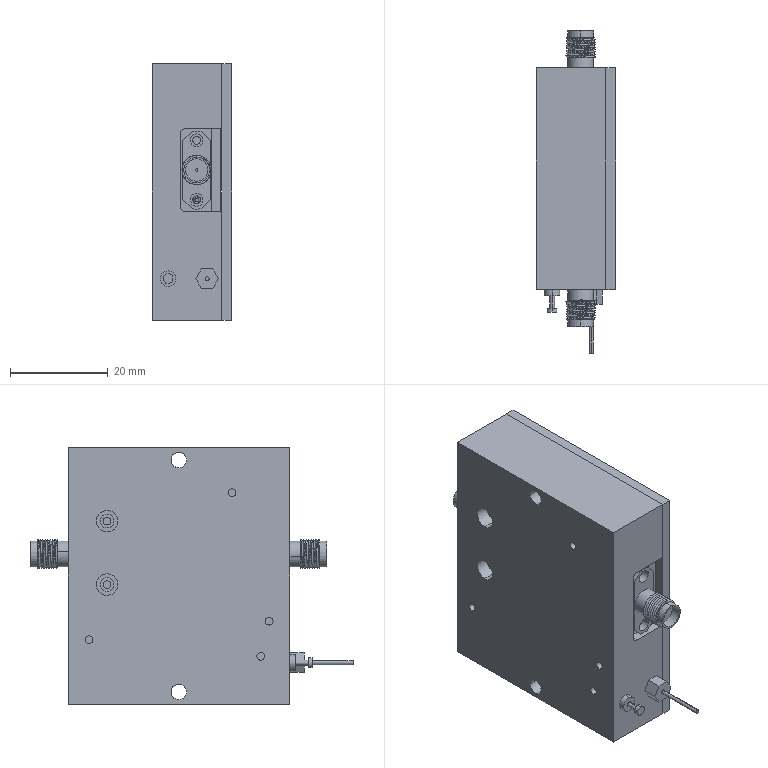CAM job | Mastercam | mm | 15 operations | part box 16.2 x 66 x 52.5
1. Facing | 20 - 63 平铣刀
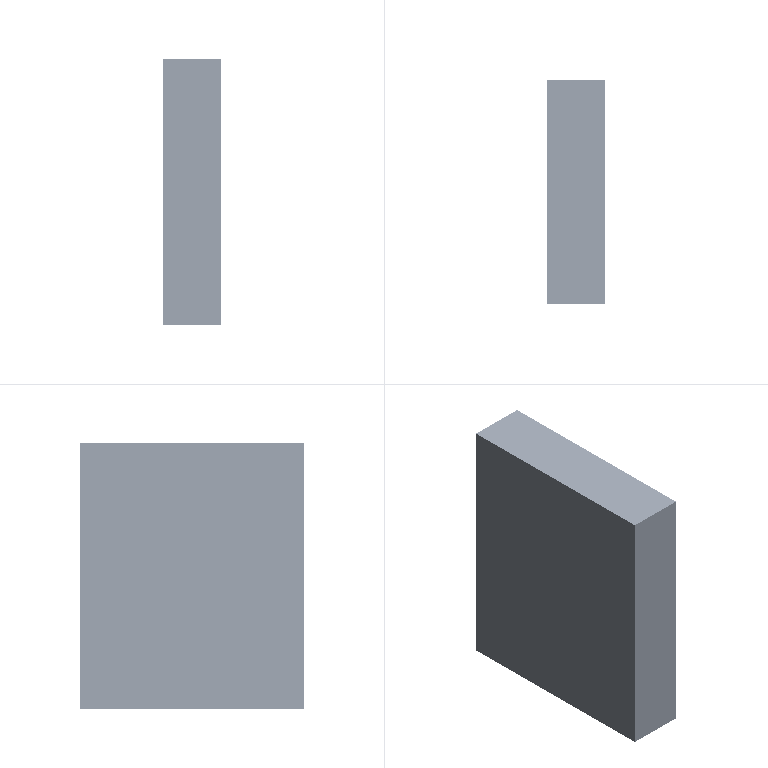2. 2D High Speed (2D Dynamic Mill) | 9 - 10 平铣刀
3. 2D High Speed (2D Area Mill) | 9 - 10 平铣刀
4. Contour (Ramp) | 18 - 10 圆鼻铣刀
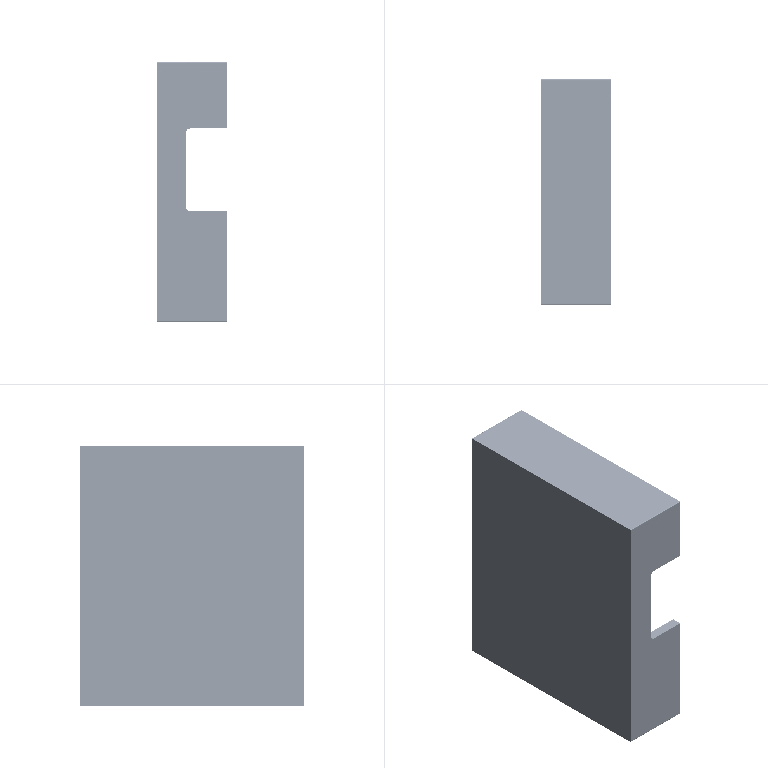5. Contour (2D) | 18 - 10 圆鼻铣刀
6. Contour (2D) | 10 - 10 平铣刀
7. Contour (Remachining) | 4 - 4 平铣刀
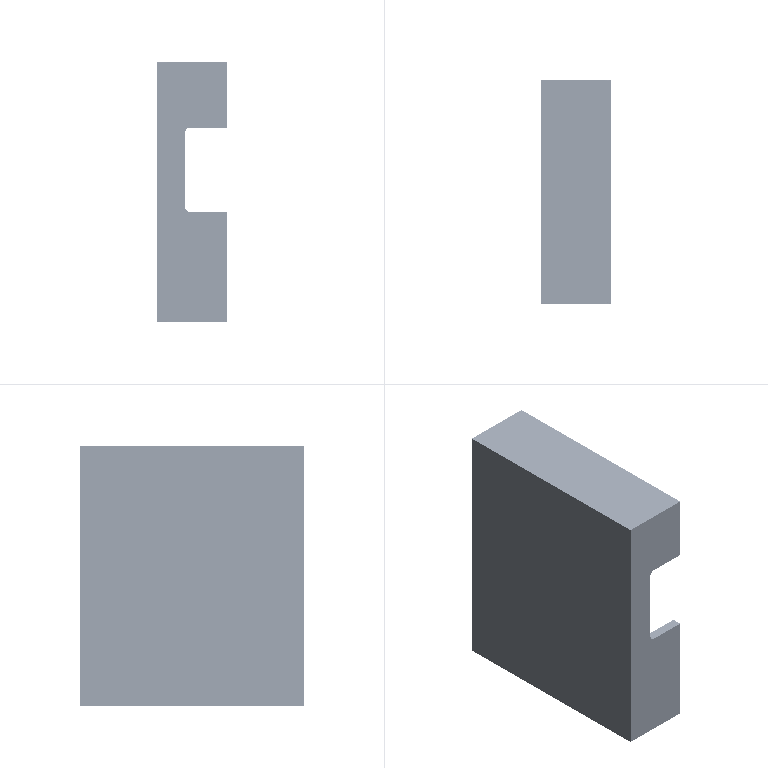8. 2D High Speed (2D Area Mill) | 4 - 4 平铣刀
9. Contour (2D) | 4 - 4 平铣刀
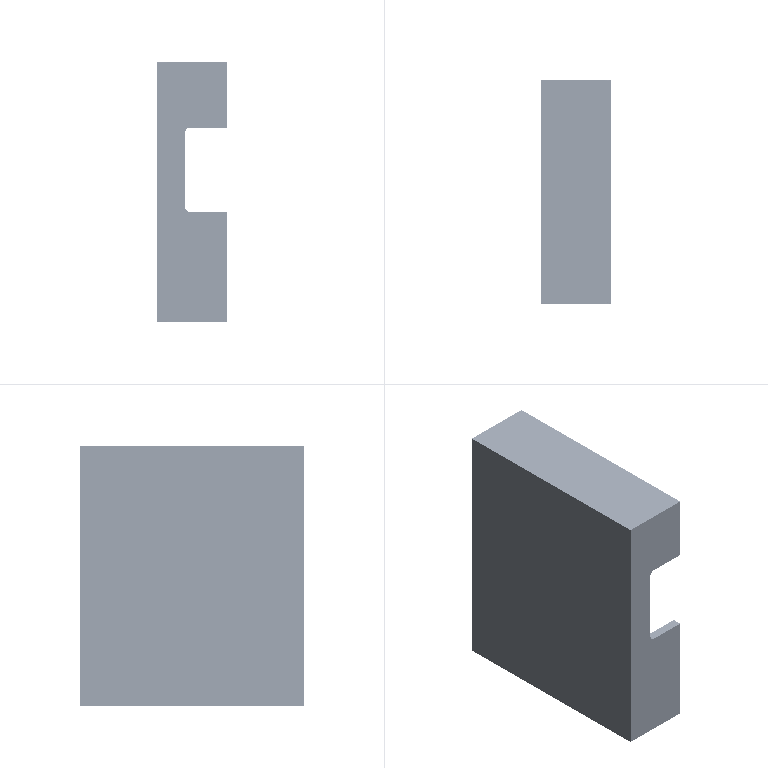10. Drill/Counterbore | 7 - 4 倒角刀
11. Deburr 5-axis Deburr 5-axis | 19 - 3 球刀/圆鼻铣刀
12. Facing | 20 - 63 平铣刀
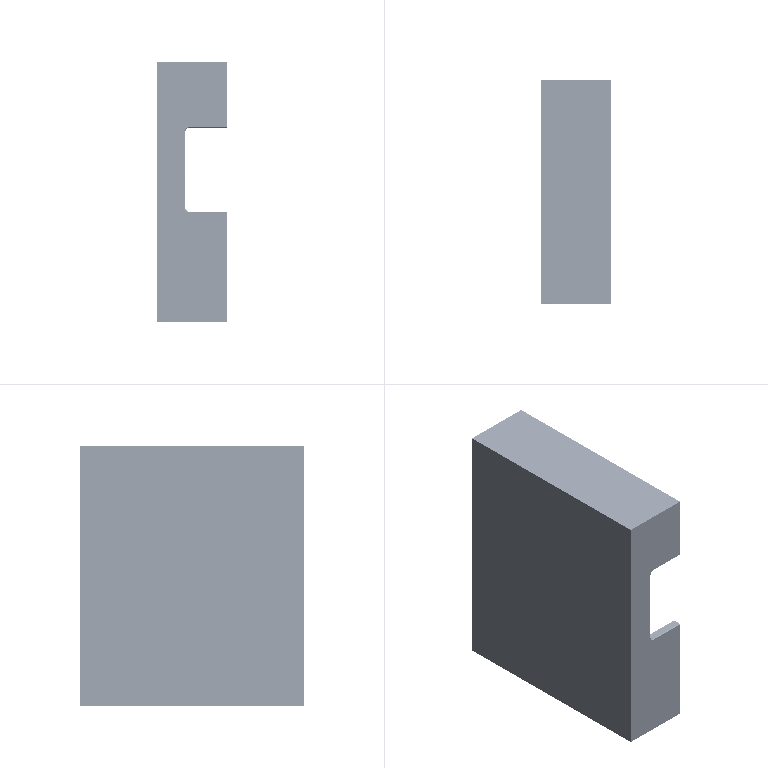13. Helix Bore | 3 - 3 平铣刀
14. Contour (2D chamfer) | 7 - 4 倒角刀
15. Drill/Counterbore | 7 - 4 倒角刀